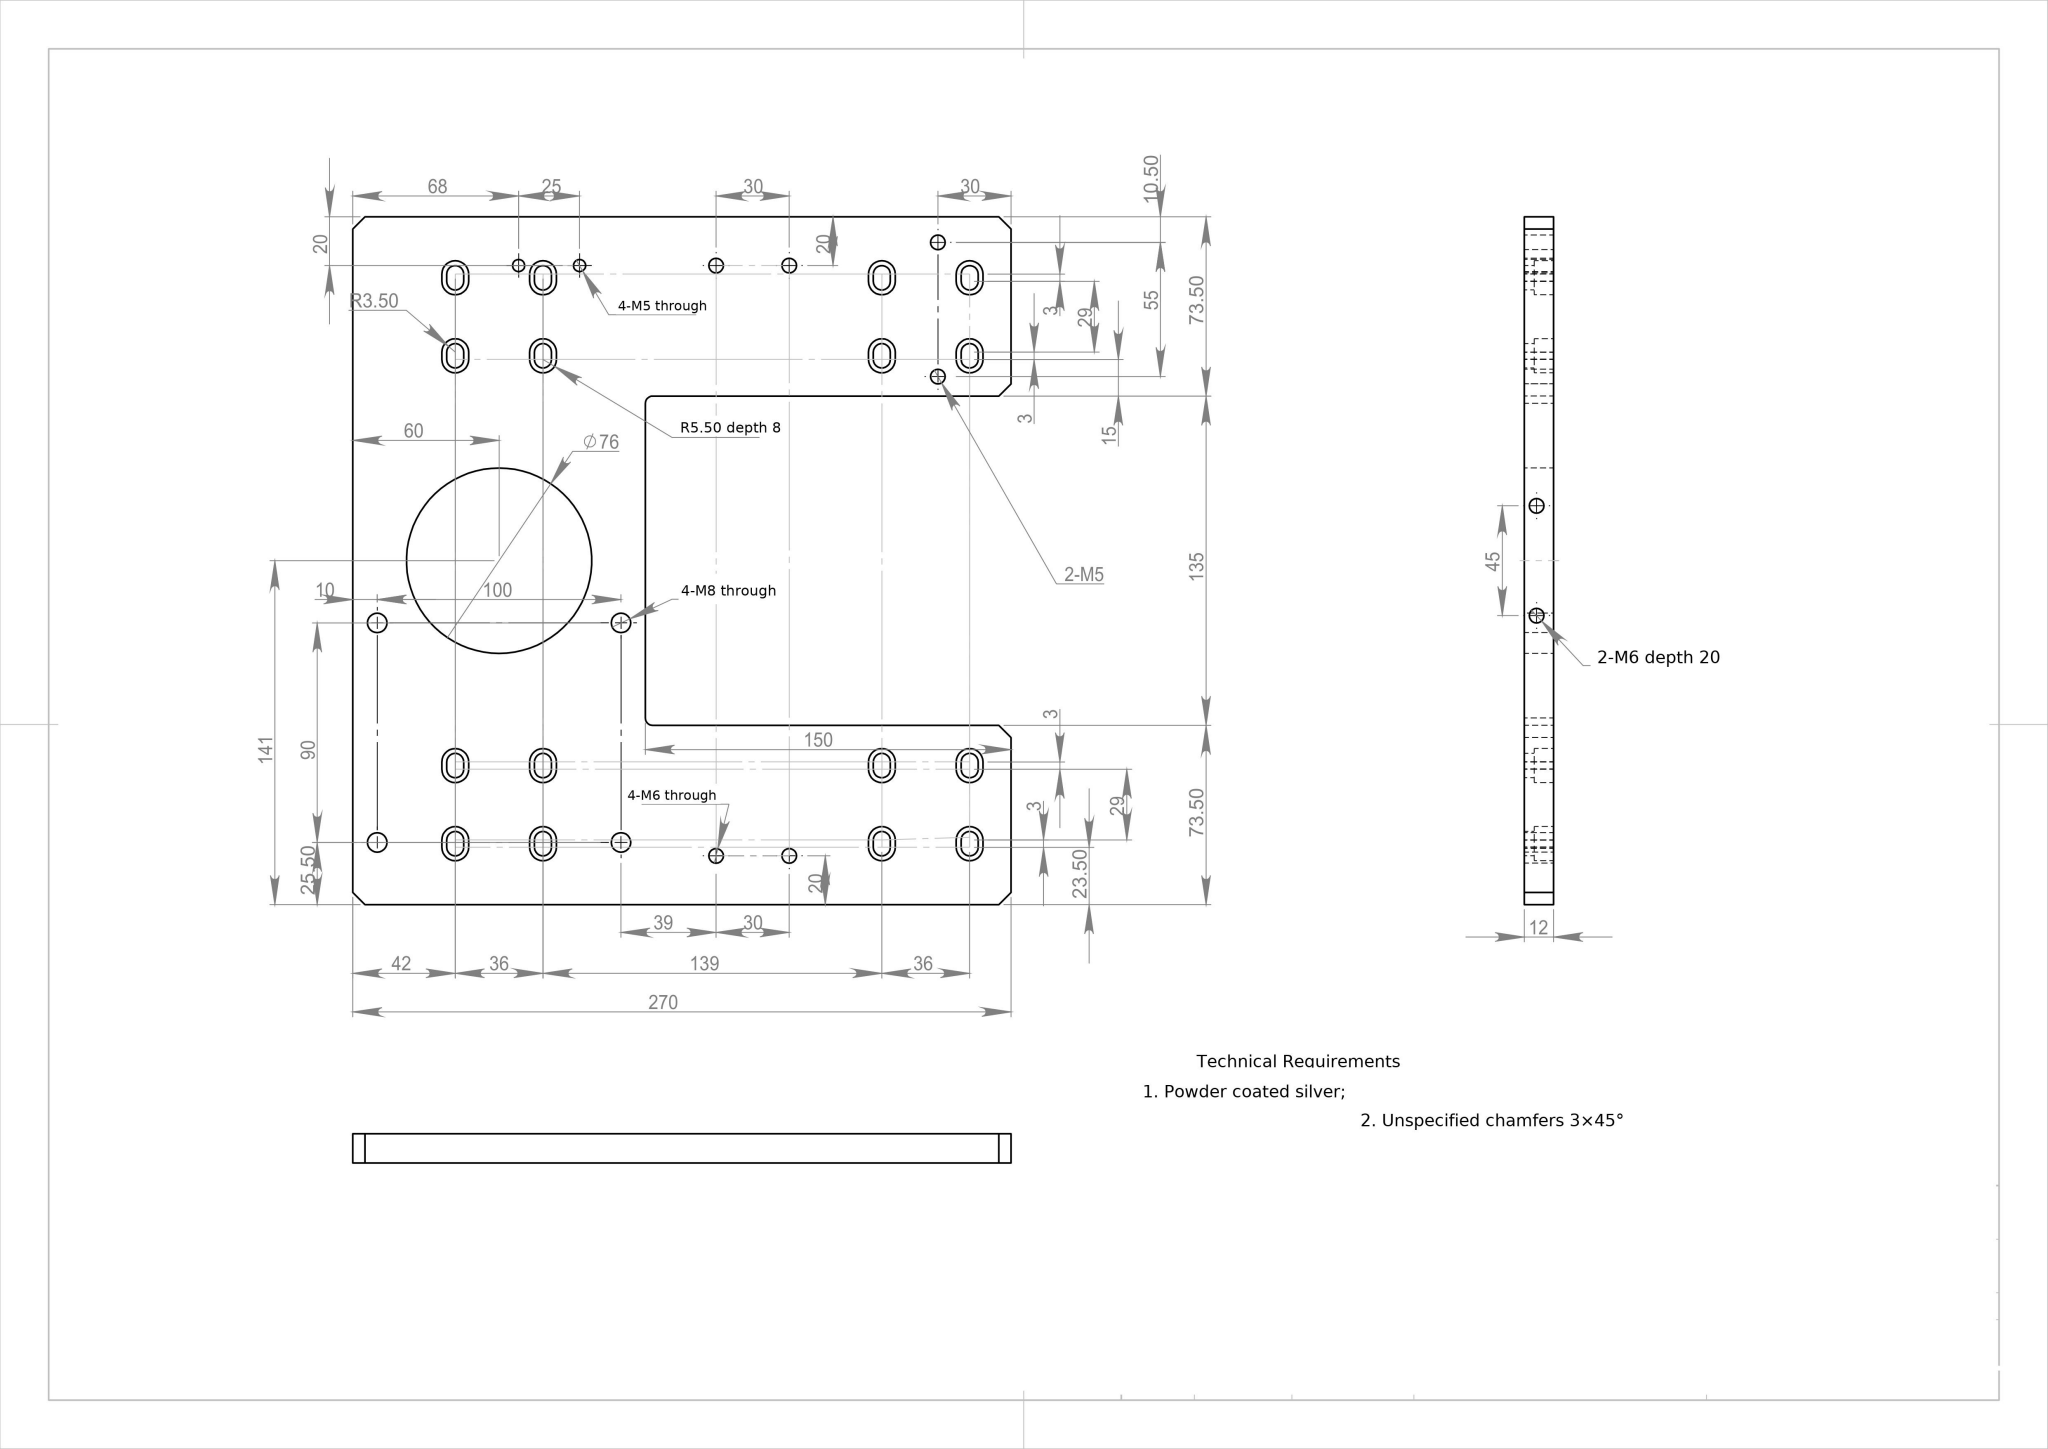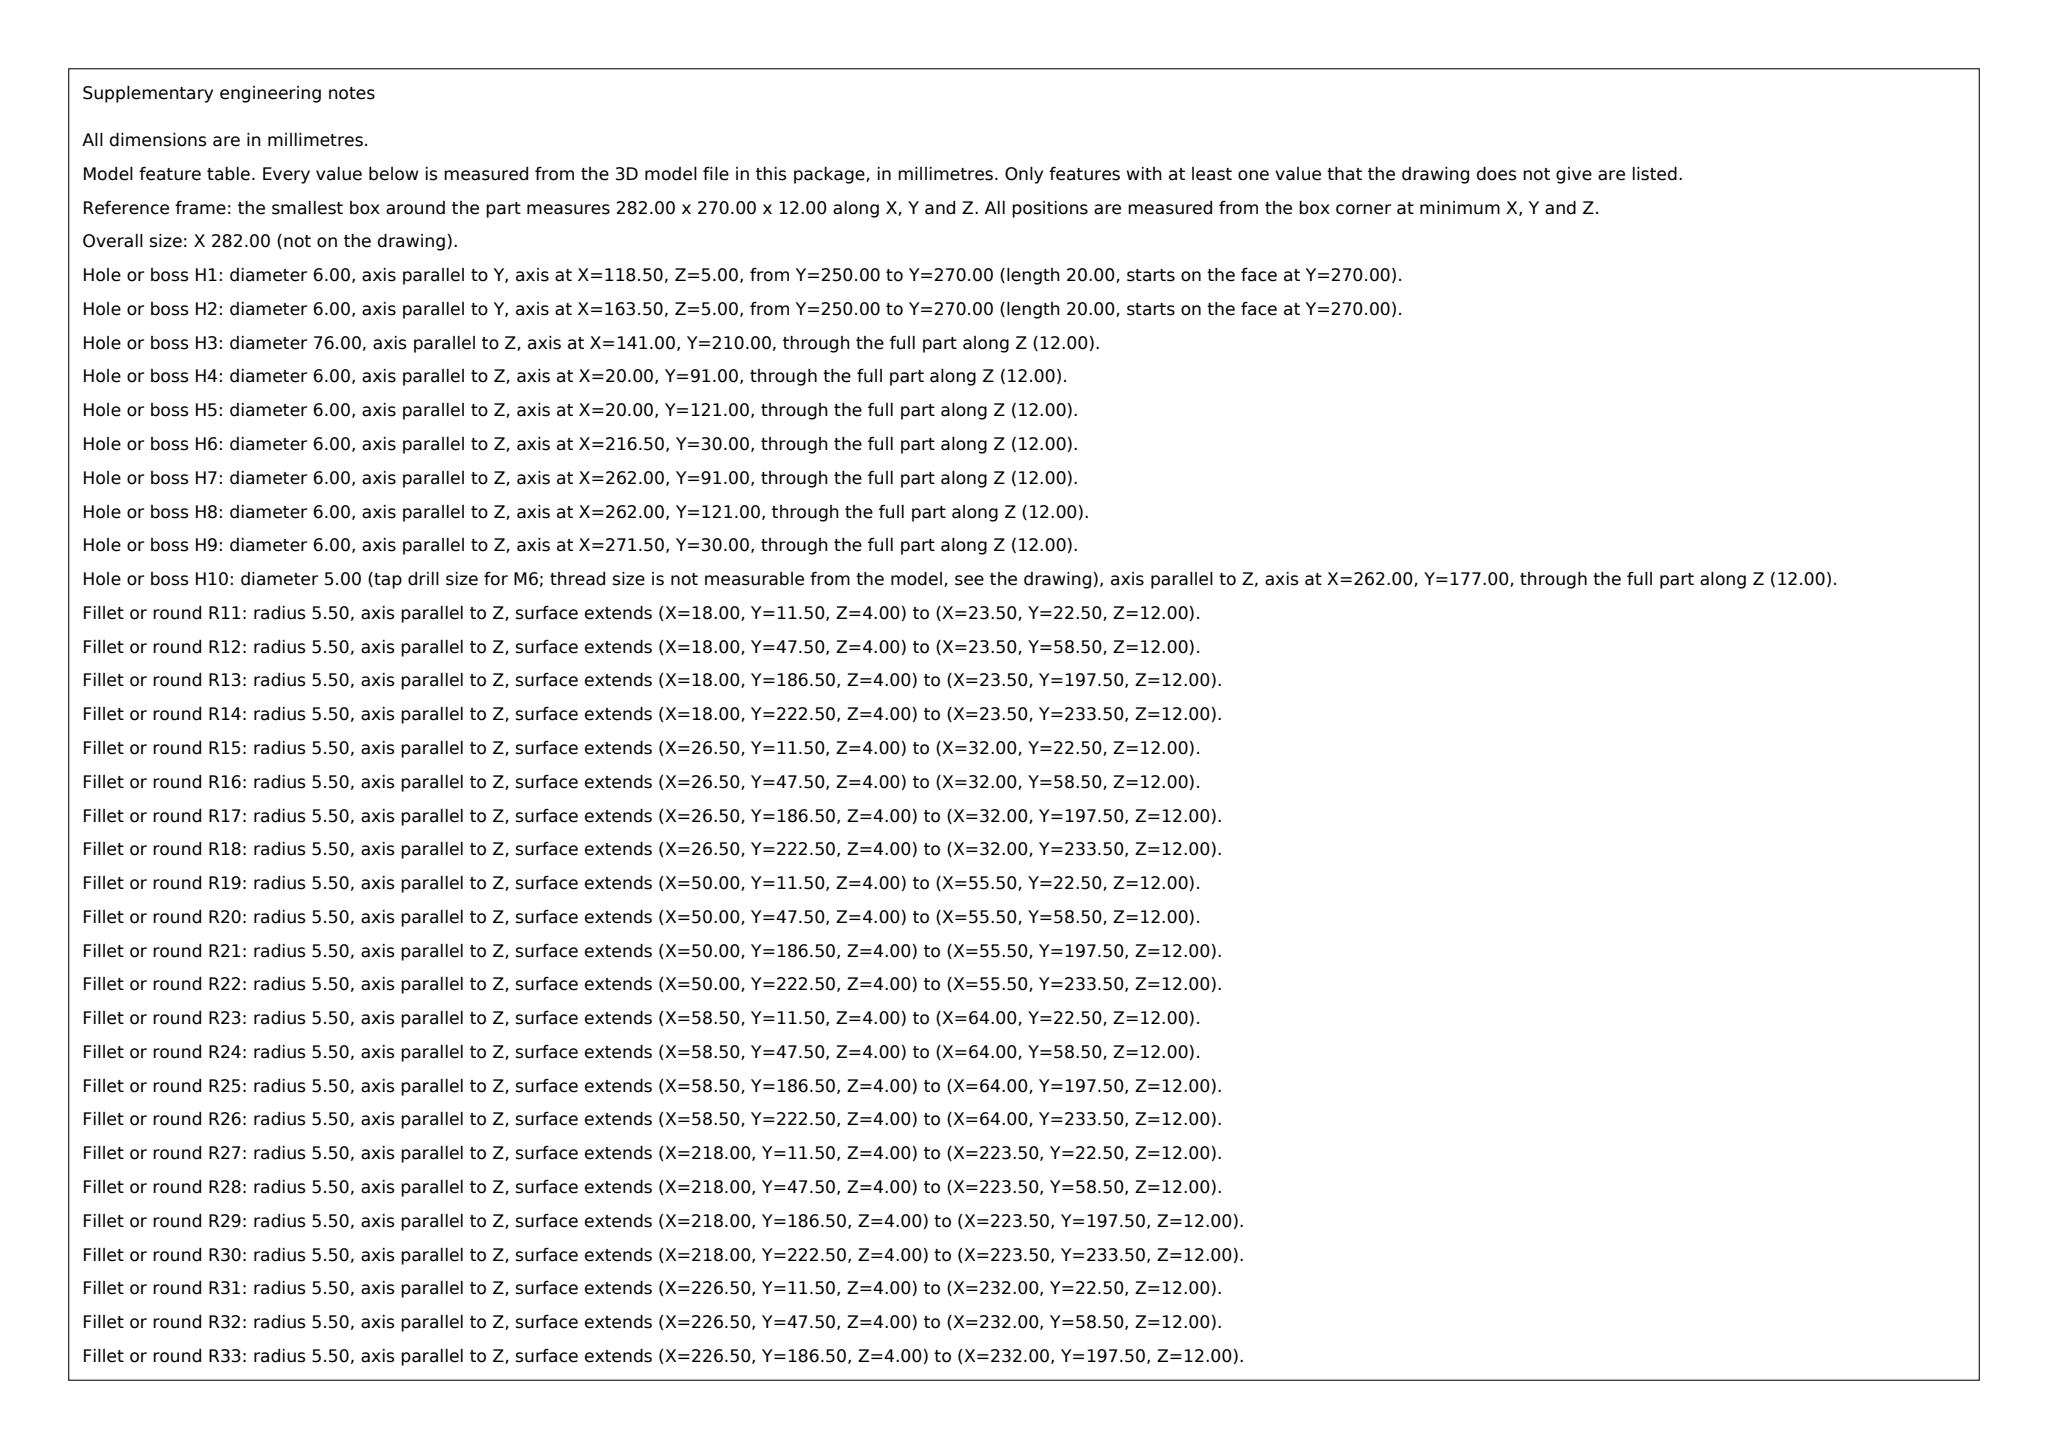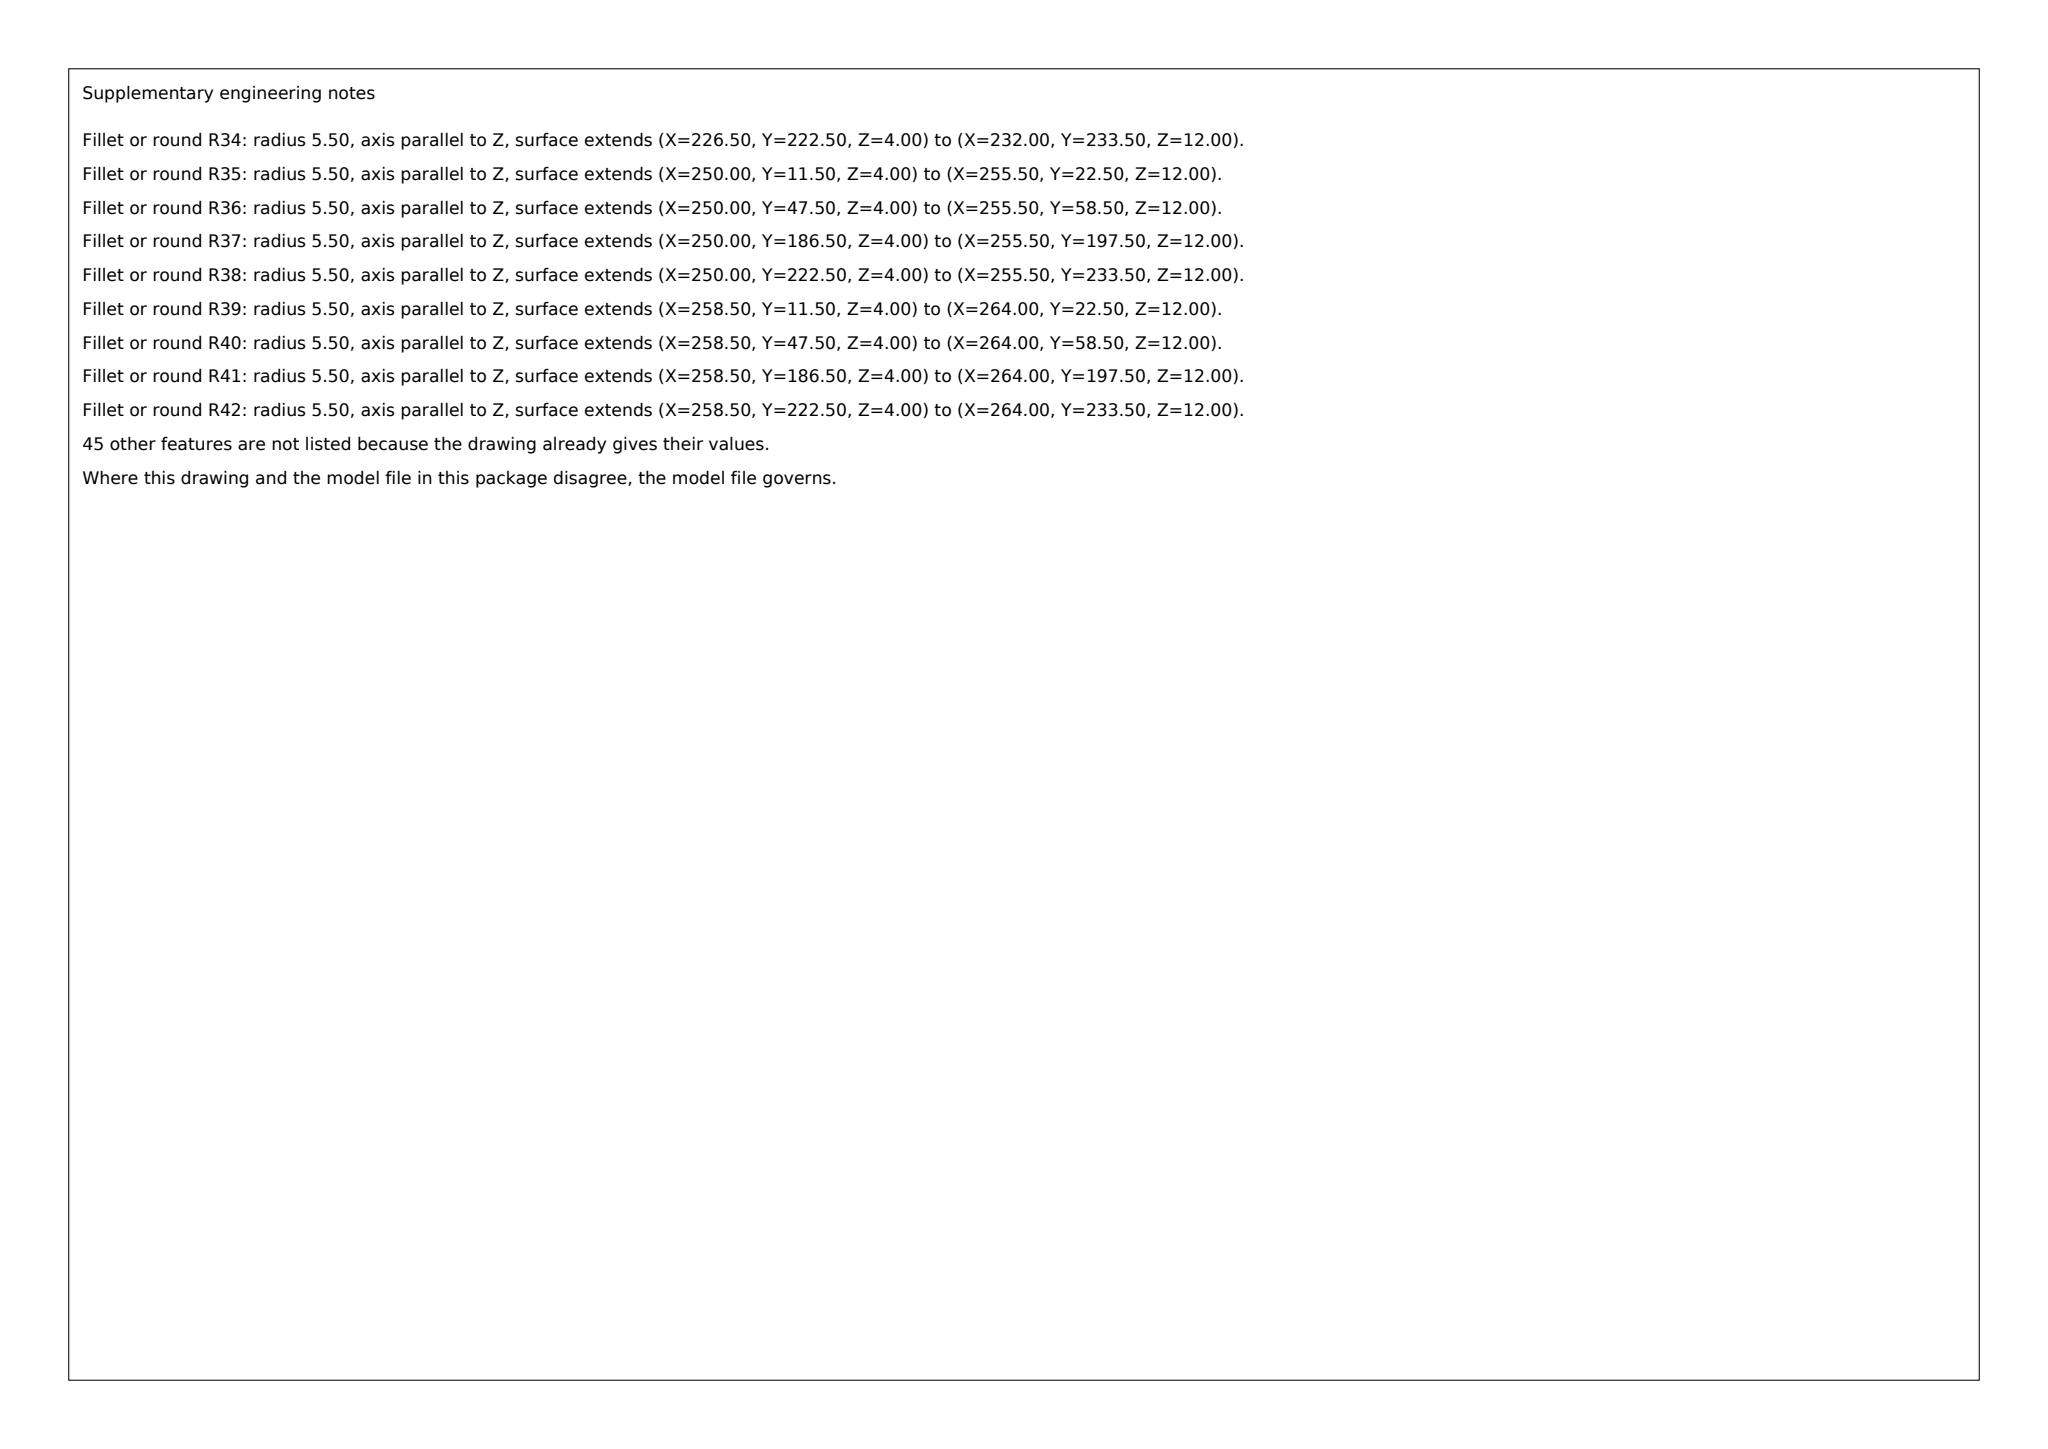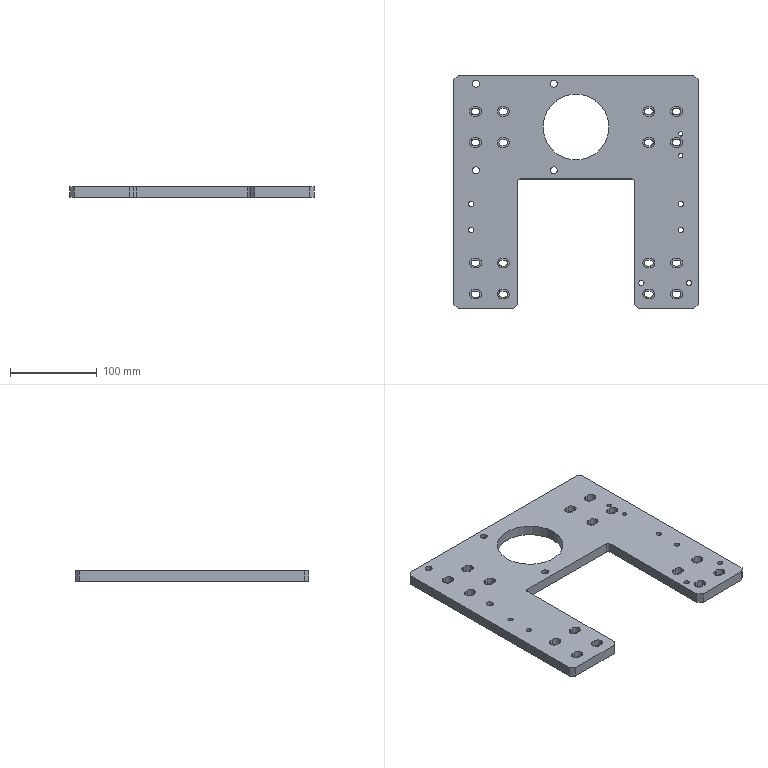Part | SolidWorks | mm | 1 solid | 227 faces | box 282 x 270 x 12 mm | volume 589263 mm3 | cylinder 129 | plane 98 | commonest cylinder face diameters 11 x48 7 x48 6 x19 8 x8 5 x4 76 x2
build123d program:
from build123d import *

# Parameters (mm, degrees)
SKETCH1_W               = 282
SKETCH1_H               = 120
BOSS_EXTRUDE1_DEPTH     = 12
CUT_EXTRUDE1_DEPTH      = 154.704
CUT_EXTRUDE2_DEPTH      = 8
LPATTERN1_COUNT         = 2
LPATTERN1_PITCH         = 32
MIRROR1_COPY_1_DEPTH    = 154.704
MIRROR1_COPY_2_DEPTH    = 8
MIRROR2_COPY_1_DEPTH    = 154.704
MIRROR2_COPY_2_DEPTH    = 8
MIRROR2_COPY_3_DEPTH    = 154.704
MIRROR2_COPY_4_DEPTH    = 8
MIRROR2_COPY_5_DEPTH    = 154.704
MIRROR2_COPY_6_DEPTH    = 8
SKETCH4_R               = 38
CUT_EXTRUDE3_DEPTH      = 154.704
SKETCH6_W               = 282
SKETCH6_H               = 12
BOSS_EXTRUDE2_DEPTH     = 150
SKETCH7_W               = 135
SKETCH7_H               = 150
CUT_EXTRUDE4_DEPTH      = 254.229
FILLET1_R               = 3
CHAMFER1_SIZE           = 5
SKETCH8_R               = 3
CUT_EXTRUDE5_DEPTH      = 20
SKETCH10_R              = 2.5
CUT_EXTRUDE7_DEPTH      = 254.229
SKETCH11_R              = 4
CUT_EXTRUDE8_DEPTH      = 254.229
LPATTERN2_COUNT         = 2
LPATTERN2_PITCH         = 100
LPATTERN2_COUNT_DIR2    = 2
LPATTERN2_PITCH_DIR2    = 90
SKETCH12_R              = 3
CUT_EXTRUDE9_DEPTH      = 254.229
LPATTERN3_COUNT         = 2
LPATTERN3_PITCH         = 30
MIRROR4_COPY_1_SKETCH_R = 3
MIRROR4_COPY_1_DEPTH    = 254.229
SKETCH13_R              = 3
CUT_EXTRUDE10_DEPTH     = 254.229
LPATTERN4_COUNT         = 2
LPATTERN4_PITCH         = 175
LPATTERN4_COPY_1_DEPTH  = 154.704
LPATTERN4_COPY_2_DEPTH  = 8
LPATTERN4_COPY_3_DEPTH  = 154.704
LPATTERN4_COPY_4_DEPTH  = 8
LPATTERN4_COPY_5_DEPTH  = 154.704
LPATTERN4_COPY_6_DEPTH  = 8
LPATTERN4_COPY_7_DEPTH  = 154.704
LPATTERN4_COPY_8_DEPTH  = 8
LPATTERN4_COPY_9_DEPTH  = 154.704
LPATTERN4_COPY_10_DEPTH = 8
LPATTERN4_COPY_11_DEPTH = 154.704
LPATTERN4_COPY_12_DEPTH = 8
LPATTERN4_COPY_13_DEPTH = 154.704
LPATTERN4_COPY_14_DEPTH = 8
LPATTERN5_COUNT         = 2
LPATTERN5_PITCH         = 55


with BuildPart() as part:
    # Sketch1 → Boss-Extrude1 (new body)
    with BuildSketch(Plane.XY):
        Rectangle(SKETCH1_W, SKETCH1_H)
    extrude(amount=BOSS_EXTRUDE1_DEPTH)

    # Sketch2 → Cut-Extrude1 (cut, through all)
    with BuildSketch(Plane.XY.offset(12)):
        with BuildLine():
            Line((-117.5, 21.5), (-114.5, 21.5))
            ThreePointArc((-114.5, 21.5), (-111, 18), (-114.5, 14.5))
            Line((-114.5, 14.5), (-117.5, 14.5))
            ThreePointArc((-117.5, 14.5), (-121, 18), (-117.5, 21.5))
        make_face()
    cut_extrude1 = extrude(amount=-CUT_EXTRUDE1_DEPTH, mode=Mode.SUBTRACT)

    # Sketch3 → Cut-Extrude2 (cut)
    with BuildSketch(Plane.XY.offset(12)):
        with BuildLine():
            Line((-117.5, 12.5), (-114.5, 12.5))
            ThreePointArc((-114.5, 12.5), (-109, 18), (-114.5, 23.5))
            Line((-114.5, 23.5), (-117.5, 23.5))
            ThreePointArc((-117.5, 23.5), (-123, 18), (-117.5, 12.5))
        make_face()
    cut_extrude2 = extrude(amount=-CUT_EXTRUDE2_DEPTH, mode=Mode.SUBTRACT)

    # LPattern1: Cut-Extrude1, Cut-Extrude2 ×2
    with Locations(*[(i * LPATTERN1_PITCH, 0, 0) for i in range(1, LPATTERN1_COUNT)]):
        add(cut_extrude1, mode=Mode.SUBTRACT)
        add(cut_extrude2, mode=Mode.SUBTRACT)

    # Mirror1: Cut-Extrude1, Cut-Extrude2 across plane
    add(cut_extrude1.mirror(Plane.ZX), mode=Mode.SUBTRACT)
    add(cut_extrude2.mirror(Plane.ZX), mode=Mode.SUBTRACT)

    # Mirror1 copy 1 sketch → Mirror1 copy 1 (cut, through all)
    with BuildSketch(Plane(origin=(32, 0, 12), x_dir=(1, 0, 0), z_dir=(0, 0, 1))):
        with BuildLine():
            Line((-117.5, -21.5), (-114.5, -21.5))
            ThreePointArc((-114.5, -21.5), (-111, -18), (-114.5, -14.5))
            Line((-114.5, -14.5), (-117.5, -14.5))
            ThreePointArc((-117.5, -14.5), (-121, -18), (-117.5, -21.5))
        make_face()
    extrude(amount=-MIRROR1_COPY_1_DEPTH, mode=Mode.SUBTRACT)

    # Mirror1 copy 2 sketch → Mirror1 copy 2 (cut)
    with BuildSketch(Plane(origin=(32, 0, 12), x_dir=(1, 0, 0), z_dir=(0, 0, 1))):
        with BuildLine():
            Line((-117.5, -12.5), (-114.5, -12.5))
            ThreePointArc((-114.5, -12.5), (-109, -18), (-114.5, -23.5))
            Line((-114.5, -23.5), (-117.5, -23.5))
            ThreePointArc((-117.5, -23.5), (-123, -18), (-117.5, -12.5))
        make_face()
    extrude(amount=-MIRROR1_COPY_2_DEPTH, mode=Mode.SUBTRACT)

    # Mirror2: Cut-Extrude1, Cut-Extrude2 across plane
    add(cut_extrude1.mirror(Plane(origin=(0, 0, 0), x_dir=(0, 0, 1), z_dir=(1, 0, 0))), mode=Mode.SUBTRACT)
    add(cut_extrude2.mirror(Plane(origin=(0, 0, 0), x_dir=(0, 0, 1), z_dir=(1, 0, 0))), mode=Mode.SUBTRACT)

    # Mirror2 copy 1 sketch → Mirror2 copy 1 (cut, through all)
    with BuildSketch(Plane(origin=(-32, 0, 12), x_dir=(-1, 0, 0), z_dir=(0, 0, 1))):
        with BuildLine():
            Line((-117.5, -21.5), (-114.5, -21.5))
            ThreePointArc((-114.5, -21.5), (-111, -18), (-114.5, -14.5))
            Line((-114.5, -14.5), (-117.5, -14.5))
            ThreePointArc((-117.5, -14.5), (-121, -18), (-117.5, -21.5))
        make_face()
    extrude(amount=-MIRROR2_COPY_1_DEPTH, mode=Mode.SUBTRACT)

    # Mirror2 copy 2 sketch → Mirror2 copy 2 (cut)
    with BuildSketch(Plane(origin=(-32, 0, 12), x_dir=(-1, 0, 0), z_dir=(0, 0, 1))):
        with BuildLine():
            Line((-117.5, -12.5), (-114.5, -12.5))
            ThreePointArc((-114.5, -12.5), (-109, -18), (-114.5, -23.5))
            Line((-114.5, -23.5), (-117.5, -23.5))
            ThreePointArc((-117.5, -23.5), (-123, -18), (-117.5, -12.5))
        make_face()
    extrude(amount=-MIRROR2_COPY_2_DEPTH, mode=Mode.SUBTRACT)

    # Mirror2 copy 3 sketch → Mirror2 copy 3 (cut, through all)
    with BuildSketch(Plane(origin=(0, 0, 12), x_dir=(-1, 0, 0), z_dir=(0, 0, 1))):
        with BuildLine():
            Line((-117.5, 21.5), (-114.5, 21.5))
            ThreePointArc((-114.5, 21.5), (-111, 18), (-114.5, 14.5))
            Line((-114.5, 14.5), (-117.5, 14.5))
            ThreePointArc((-117.5, 14.5), (-121, 18), (-117.5, 21.5))
        make_face()
    extrude(amount=-MIRROR2_COPY_3_DEPTH, mode=Mode.SUBTRACT)

    # Mirror2 copy 4 sketch → Mirror2 copy 4 (cut)
    with BuildSketch(Plane(origin=(0, 0, 12), x_dir=(-1, 0, 0), z_dir=(0, 0, 1))):
        with BuildLine():
            Line((-117.5, 12.5), (-114.5, 12.5))
            ThreePointArc((-114.5, 12.5), (-109, 18), (-114.5, 23.5))
            Line((-114.5, 23.5), (-117.5, 23.5))
            ThreePointArc((-117.5, 23.5), (-123, 18), (-117.5, 12.5))
        make_face()
    extrude(amount=-MIRROR2_COPY_4_DEPTH, mode=Mode.SUBTRACT)

    # Mirror2 copy 5 sketch → Mirror2 copy 5 (cut, through all)
    with BuildSketch(Plane(origin=(-32, 0, 12), x_dir=(-1, 0, 0), z_dir=(0, 0, 1))):
        with BuildLine():
            Line((-117.5, 21.5), (-114.5, 21.5))
            ThreePointArc((-114.5, 21.5), (-111, 18), (-114.5, 14.5))
            Line((-114.5, 14.5), (-117.5, 14.5))
            ThreePointArc((-117.5, 14.5), (-121, 18), (-117.5, 21.5))
        make_face()
    extrude(amount=-MIRROR2_COPY_5_DEPTH, mode=Mode.SUBTRACT)

    # Mirror2 copy 6 sketch → Mirror2 copy 6 (cut)
    with BuildSketch(Plane(origin=(-32, 0, 12), x_dir=(-1, 0, 0), z_dir=(0, 0, 1))):
        with BuildLine():
            Line((-117.5, 12.5), (-114.5, 12.5))
            ThreePointArc((-114.5, 12.5), (-109, 18), (-114.5, 23.5))
            Line((-114.5, 23.5), (-117.5, 23.5))
            ThreePointArc((-117.5, 23.5), (-123, 18), (-117.5, 12.5))
        make_face()
    extrude(amount=-MIRROR2_COPY_6_DEPTH, mode=Mode.SUBTRACT)

    # Sketch4 → Cut-Extrude3 (cut, through all)
    with BuildSketch(Plane.XY.offset(12)):
        Circle(SKETCH4_R)
    extrude(amount=-CUT_EXTRUDE3_DEPTH, mode=Mode.SUBTRACT)

    # Sketch6 → Boss-Extrude2 (add)
    with BuildSketch(Plane(origin=(0, -60, 0), x_dir=(1, 0, 0), z_dir=(0, 1, 0))):
        with Locations((0, -6)):
            Rectangle(SKETCH6_W, SKETCH6_H)
    extrude(amount=-BOSS_EXTRUDE2_DEPTH)

    # Sketch7 → Cut-Extrude4 (cut, through all)
    with BuildSketch(Plane(origin=(0, 0, 0), x_dir=(-1, 0, 0), z_dir=(0, 0, -1))):
        with Locations((0, -135)):
            Rectangle(SKETCH7_W, SKETCH7_H)
    extrude(amount=-CUT_EXTRUDE4_DEPTH, mode=Mode.SUBTRACT)

    # Fillet1
    fillet1_edges = [part.edges().sort_by_distance(p)[0] for p in [
        (67.5, -60, 6),
        (-67.5, -60, 6),
    ]]
    fillet(fillet1_edges, radius=FILLET1_R)

    # Chamfer1
    chamfer1_edges = [part.edges().sort_by_distance(p)[0] for p in [
        (-141, -210, 6),
        (141, -210, 6),
        (67.5, -210, 6),
        (-67.5, -210, 6),
        (-141, 60, 6),
        (141, 60, 6),
    ]]
    chamfer(chamfer1_edges, length=CHAMFER1_SIZE)

    # Sketch8 → Cut-Extrude5 (cut)
    with BuildSketch(Plane(origin=(0, 60, 0), x_dir=(1, 0, 0), z_dir=(0, 1, 0))):
        with Locations(Location((-22.5, -5, 0), (0, 0, 270))):
            Circle(SKETCH8_R)
    cut_extrude5 = extrude(amount=-CUT_EXTRUDE5_DEPTH, mode=Mode.SUBTRACT)

    # Mirror3: Cut-Extrude5 across plane
    add(cut_extrude5.mirror(Plane(origin=(0, 0, 0), x_dir=(0, 0, 1), z_dir=(1, 0, 0))), mode=Mode.SUBTRACT)

    # Sketch10 → Cut-Extrude7 (cut, through all)
    with BuildSketch(Plane.XY.offset(12)):
        with Locations((121, -8)):
            Circle(SKETCH10_R)
        with Locations((121, -33)):
            Circle(SKETCH10_R)
    extrude(amount=-CUT_EXTRUDE7_DEPTH, mode=Mode.SUBTRACT)

    # Sketch11 → Cut-Extrude8 (cut, through all)
    with BuildSketch(Plane.XY.offset(12)):
        with Locations((-115.5, 50)):
            Circle(SKETCH11_R)
    cut_extrude8 = extrude(amount=-CUT_EXTRUDE8_DEPTH, mode=Mode.SUBTRACT)

    # LPattern2: Cut-Extrude8 2 × 2
    with Locations(*[(j * LPATTERN2_PITCH_DIR2, -i * LPATTERN2_PITCH, 0) for i in range(LPATTERN2_COUNT) for j in range(LPATTERN2_COUNT_DIR2) if (i, j) != (0, 0)]):
        add(cut_extrude8, mode=Mode.SUBTRACT)

    # Sketch12 → Cut-Extrude9 (cut, through all)
    with BuildSketch(Plane.XY.offset(12)):
        with Locations((-121, -119)):
            Circle(SKETCH12_R)
    cut_extrude9 = extrude(amount=-CUT_EXTRUDE9_DEPTH, mode=Mode.SUBTRACT)

    # LPattern3: Cut-Extrude9 ×2
    with Locations(*[(0, i * LPATTERN3_PITCH, 0) for i in range(1, LPATTERN3_COUNT)]):
        add(cut_extrude9, mode=Mode.SUBTRACT)

    # Mirror4: Cut-Extrude9 across plane
    add(cut_extrude9.mirror(Plane(origin=(0, 0, 0), x_dir=(0, 0, 1), z_dir=(1, 0, 0))), mode=Mode.SUBTRACT)

    # Mirror4 copy 1 sketch → Mirror4 copy 1 (cut, through all)
    with BuildSketch(Plane(origin=(0, 30, 12), x_dir=(-1, 0, 0), z_dir=(0, 0, 1))):
        with Locations((-121, 119)):
            Circle(MIRROR4_COPY_1_SKETCH_R)
    extrude(amount=-MIRROR4_COPY_1_DEPTH, mode=Mode.SUBTRACT)

    # Sketch13 → Cut-Extrude10 (cut, through all)
    with BuildSketch(Plane.XY.offset(12)):
        with Locations((75.5, -180)):
            Circle(SKETCH13_R)
    cut_extrude10 = extrude(amount=-CUT_EXTRUDE10_DEPTH, mode=Mode.SUBTRACT)

    # LPattern4: Cut-Extrude1, Cut-Extrude2 ×2
    with Locations(*[(0, -i * LPATTERN4_PITCH, 0) for i in range(1, LPATTERN4_COUNT)]):
        add(cut_extrude1, mode=Mode.SUBTRACT)
        add(cut_extrude2, mode=Mode.SUBTRACT)

    # LPattern4 copy 1 sketch → LPattern4 copy 1 (cut, through all)
    with BuildSketch(Plane(origin=(32, -175, 12), x_dir=(1, 0, 0), z_dir=(0, 0, 1))):
        with BuildLine():
            Line((-117.5, 21.5), (-114.5, 21.5))
            ThreePointArc((-114.5, 21.5), (-111, 18), (-114.5, 14.5))
            Line((-114.5, 14.5), (-117.5, 14.5))
            ThreePointArc((-117.5, 14.5), (-121, 18), (-117.5, 21.5))
        make_face()
    extrude(amount=-LPATTERN4_COPY_1_DEPTH, mode=Mode.SUBTRACT)

    # LPattern4 copy 2 sketch → LPattern4 copy 2 (cut)
    with BuildSketch(Plane(origin=(32, -175, 12), x_dir=(1, 0, 0), z_dir=(0, 0, 1))):
        with BuildLine():
            Line((-117.5, 12.5), (-114.5, 12.5))
            ThreePointArc((-114.5, 12.5), (-109, 18), (-114.5, 23.5))
            Line((-114.5, 23.5), (-117.5, 23.5))
            ThreePointArc((-117.5, 23.5), (-123, 18), (-117.5, 12.5))
        make_face()
    extrude(amount=-LPATTERN4_COPY_2_DEPTH, mode=Mode.SUBTRACT)

    # LPattern4 copy 3 sketch → LPattern4 copy 3 (cut, through all)
    with BuildSketch(Plane(origin=(0, -175, 12), x_dir=(1, 0, 0), z_dir=(0, 0, 1))):
        with BuildLine():
            Line((-117.5, -21.5), (-114.5, -21.5))
            ThreePointArc((-114.5, -21.5), (-111, -18), (-114.5, -14.5))
            Line((-114.5, -14.5), (-117.5, -14.5))
            ThreePointArc((-117.5, -14.5), (-121, -18), (-117.5, -21.5))
        make_face()
    extrude(amount=-LPATTERN4_COPY_3_DEPTH, mode=Mode.SUBTRACT)

    # LPattern4 copy 4 sketch → LPattern4 copy 4 (cut)
    with BuildSketch(Plane(origin=(0, -175, 12), x_dir=(1, 0, 0), z_dir=(0, 0, 1))):
        with BuildLine():
            Line((-117.5, -12.5), (-114.5, -12.5))
            ThreePointArc((-114.5, -12.5), (-109, -18), (-114.5, -23.5))
            Line((-114.5, -23.5), (-117.5, -23.5))
            ThreePointArc((-117.5, -23.5), (-123, -18), (-117.5, -12.5))
        make_face()
    extrude(amount=-LPATTERN4_COPY_4_DEPTH, mode=Mode.SUBTRACT)

    # LPattern4 copy 5 sketch → LPattern4 copy 5 (cut, through all)
    with BuildSketch(Plane(origin=(32, -175, 12), x_dir=(1, 0, 0), z_dir=(0, 0, 1))):
        with BuildLine():
            Line((-117.5, -21.5), (-114.5, -21.5))
            ThreePointArc((-114.5, -21.5), (-111, -18), (-114.5, -14.5))
            Line((-114.5, -14.5), (-117.5, -14.5))
            ThreePointArc((-117.5, -14.5), (-121, -18), (-117.5, -21.5))
        make_face()
    extrude(amount=-LPATTERN4_COPY_5_DEPTH, mode=Mode.SUBTRACT)

    # LPattern4 copy 6 sketch → LPattern4 copy 6 (cut)
    with BuildSketch(Plane(origin=(32, -175, 12), x_dir=(1, 0, 0), z_dir=(0, 0, 1))):
        with BuildLine():
            Line((-117.5, -12.5), (-114.5, -12.5))
            ThreePointArc((-114.5, -12.5), (-109, -18), (-114.5, -23.5))
            Line((-114.5, -23.5), (-117.5, -23.5))
            ThreePointArc((-117.5, -23.5), (-123, -18), (-117.5, -12.5))
        make_face()
    extrude(amount=-LPATTERN4_COPY_6_DEPTH, mode=Mode.SUBTRACT)

    # LPattern4 copy 7 sketch → LPattern4 copy 7 (cut, through all)
    with BuildSketch(Plane(origin=(0, -175, 12), x_dir=(-1, 0, 0), z_dir=(0, 0, 1))):
        with BuildLine():
            Line((-117.5, -21.5), (-114.5, -21.5))
            ThreePointArc((-114.5, -21.5), (-111, -18), (-114.5, -14.5))
            Line((-114.5, -14.5), (-117.5, -14.5))
            ThreePointArc((-117.5, -14.5), (-121, -18), (-117.5, -21.5))
        make_face()
    extrude(amount=-LPATTERN4_COPY_7_DEPTH, mode=Mode.SUBTRACT)

    # LPattern4 copy 8 sketch → LPattern4 copy 8 (cut)
    with BuildSketch(Plane(origin=(0, -175, 12), x_dir=(-1, 0, 0), z_dir=(0, 0, 1))):
        with BuildLine():
            Line((-117.5, -12.5), (-114.5, -12.5))
            ThreePointArc((-114.5, -12.5), (-109, -18), (-114.5, -23.5))
            Line((-114.5, -23.5), (-117.5, -23.5))
            ThreePointArc((-117.5, -23.5), (-123, -18), (-117.5, -12.5))
        make_face()
    extrude(amount=-LPATTERN4_COPY_8_DEPTH, mode=Mode.SUBTRACT)

    # LPattern4 copy 9 sketch → LPattern4 copy 9 (cut, through all)
    with BuildSketch(Plane(origin=(-32, -175, 12), x_dir=(-1, 0, 0), z_dir=(0, 0, 1))):
        with BuildLine():
            Line((-117.5, -21.5), (-114.5, -21.5))
            ThreePointArc((-114.5, -21.5), (-111, -18), (-114.5, -14.5))
            Line((-114.5, -14.5), (-117.5, -14.5))
            ThreePointArc((-117.5, -14.5), (-121, -18), (-117.5, -21.5))
        make_face()
    extrude(amount=-LPATTERN4_COPY_9_DEPTH, mode=Mode.SUBTRACT)

    # LPattern4 copy 10 sketch → LPattern4 copy 10 (cut)
    with BuildSketch(Plane(origin=(-32, -175, 12), x_dir=(-1, 0, 0), z_dir=(0, 0, 1))):
        with BuildLine():
            Line((-117.5, -12.5), (-114.5, -12.5))
            ThreePointArc((-114.5, -12.5), (-109, -18), (-114.5, -23.5))
            Line((-114.5, -23.5), (-117.5, -23.5))
            ThreePointArc((-117.5, -23.5), (-123, -18), (-117.5, -12.5))
        make_face()
    extrude(amount=-LPATTERN4_COPY_10_DEPTH, mode=Mode.SUBTRACT)

    # LPattern4 copy 11 sketch → LPattern4 copy 11 (cut, through all)
    with BuildSketch(Plane(origin=(0, -175, 12), x_dir=(-1, 0, 0), z_dir=(0, 0, 1))):
        with BuildLine():
            Line((-117.5, 21.5), (-114.5, 21.5))
            ThreePointArc((-114.5, 21.5), (-111, 18), (-114.5, 14.5))
            Line((-114.5, 14.5), (-117.5, 14.5))
            ThreePointArc((-117.5, 14.5), (-121, 18), (-117.5, 21.5))
        make_face()
    extrude(amount=-LPATTERN4_COPY_11_DEPTH, mode=Mode.SUBTRACT)

    # LPattern4 copy 12 sketch → LPattern4 copy 12 (cut)
    with BuildSketch(Plane(origin=(0, -175, 12), x_dir=(-1, 0, 0), z_dir=(0, 0, 1))):
        with BuildLine():
            Line((-117.5, 12.5), (-114.5, 12.5))
            ThreePointArc((-114.5, 12.5), (-109, 18), (-114.5, 23.5))
            Line((-114.5, 23.5), (-117.5, 23.5))
            ThreePointArc((-117.5, 23.5), (-123, 18), (-117.5, 12.5))
        make_face()
    extrude(amount=-LPATTERN4_COPY_12_DEPTH, mode=Mode.SUBTRACT)

    # LPattern4 copy 13 sketch → LPattern4 copy 13 (cut, through all)
    with BuildSketch(Plane(origin=(-32, -175, 12), x_dir=(-1, 0, 0), z_dir=(0, 0, 1))):
        with BuildLine():
            Line((-117.5, 21.5), (-114.5, 21.5))
            ThreePointArc((-114.5, 21.5), (-111, 18), (-114.5, 14.5))
            Line((-114.5, 14.5), (-117.5, 14.5))
            ThreePointArc((-117.5, 14.5), (-121, 18), (-117.5, 21.5))
        make_face()
    extrude(amount=-LPATTERN4_COPY_13_DEPTH, mode=Mode.SUBTRACT)

    # LPattern4 copy 14 sketch → LPattern4 copy 14 (cut)
    with BuildSketch(Plane(origin=(-32, -175, 12), x_dir=(-1, 0, 0), z_dir=(0, 0, 1))):
        with BuildLine():
            Line((-117.5, 12.5), (-114.5, 12.5))
            ThreePointArc((-114.5, 12.5), (-109, 18), (-114.5, 23.5))
            Line((-114.5, 23.5), (-117.5, 23.5))
            ThreePointArc((-117.5, 23.5), (-123, 18), (-117.5, 12.5))
        make_face()
    extrude(amount=-LPATTERN4_COPY_14_DEPTH, mode=Mode.SUBTRACT)

    # LPattern5: Cut-Extrude10 ×2
    with Locations(*[(i * LPATTERN5_PITCH, 0, 0) for i in range(1, LPATTERN5_COUNT)]):
        add(cut_extrude10, mode=Mode.SUBTRACT)


solid = part.part